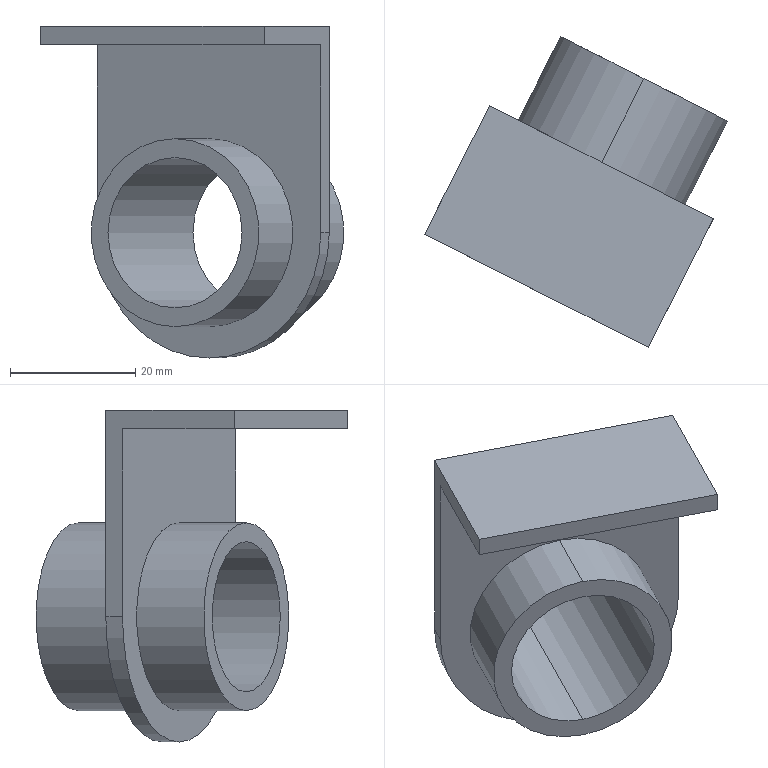Component | SolidWorks | ScribingMechanismAssembly-1_ScribingPlateFixedSleeve-1 | 1 solid | 17 faces | box 48.4 x 49.72 x 53 mm | volume 13758 mm3 | plane 9 | cylinder 8 | commonest cylinder face diameters 30 x4 24 x2 40 x2
STEP:
#1=COLOUR_RGB('',0.7922,0.8196,0.9333);
#2=FILL_AREA_STYLE_COLOUR('',#1);
#3=FILL_AREA_STYLE('',(#2));
#4=SURFACE_STYLE_FILL_AREA(#3);
#5=SURFACE_SIDE_STYLE('',(#4));
#6=SURFACE_STYLE_USAGE(.BOTH.,#5);
#7=PRESENTATION_STYLE_ASSIGNMENT((#6));
#8=CARTESIAN_POINT('',(-11.093,-16.169,37.952));
#9=VERTEX_POINT('',#8);
#10=CARTESIAN_POINT('',(-11.093,-16.169,36.771));
#11=VERTEX_POINT('',#10);
#12=CARTESIAN_POINT('',(-11.093,-16.169,37.361));
#13=DIRECTION('',(0.4521,0.892,0.));
#14=DIRECTION('',(-0.,-0.,1.));
#15=AXIS2_PLACEMENT_3D('',#12,#13,#14);
#16=CIRCLE('',#15,0.5906);
#17=EDGE_CURVE('',#9,#11,#16,.T.);
#18=ORIENTED_EDGE('',*,*,#17,.F.);
#19=CARTESIAN_POINT('',(-11.36,-16.696,37.952));
#20=VERTEX_POINT('',#19);
#21=CARTESIAN_POINT('',(-11.093,-16.169,37.952));
#22=DIRECTION('',(-0.4521,-0.892,-0.));
#23=VECTOR('',#22,39.37);
#24=LINE('',#21,#23);
#25=EDGE_CURVE('',#9,#20,#24,.T.);
#26=ORIENTED_EDGE('',*,*,#25,.T.);
#27=CARTESIAN_POINT('',(-11.36,-16.696,36.771));
#28=VERTEX_POINT('',#27);
#29=CARTESIAN_POINT('',(-11.36,-16.696,37.361));
#30=DIRECTION('',(-0.4521,-0.892,-0.));
#31=DIRECTION('',(0.892,-0.4521,-0.));
#32=AXIS2_PLACEMENT_3D('',#29,#30,#31);
#33=CIRCLE('',#32,0.5906);
#34=EDGE_CURVE('',#28,#20,#33,.T.);
#35=ORIENTED_EDGE('',*,*,#34,.F.);
#36=CARTESIAN_POINT('',(-11.093,-16.169,36.771));
#37=DIRECTION('',(-0.4521,-0.892,-0.));
#38=VECTOR('',#37,39.37);
#39=LINE('',#36,#38);
#40=EDGE_CURVE('',#11,#28,#39,.T.);
#41=ORIENTED_EDGE('',*,*,#40,.F.);
#42=EDGE_LOOP('',(#18,#26,#35,#41));
#43=FACE_OUTER_BOUND('',#42,.T.);
#44=CARTESIAN_POINT('',(-11.093,-16.169,37.361));
#45=DIRECTION('',(-0.4521,-0.892,-0.));
#46=DIRECTION('',(0.,0.,-1.));
#47=AXIS2_PLACEMENT_3D('',#44,#45,#46);
#48=CYLINDRICAL_SURFACE('',#47,0.5906);
#49=ADVANCED_FACE('',(#43),#48,.T.);
#50=CARTESIAN_POINT('',(-11.627,-17.223,36.889));
#51=VERTEX_POINT('',#50);
#52=CARTESIAN_POINT('',(-11.627,-17.223,37.834));
#53=VERTEX_POINT('',#52);
#54=CARTESIAN_POINT('',(-11.627,-17.223,37.361));
#55=DIRECTION('',(0.4521,0.892,0.));
#56=DIRECTION('',(-0.,-0.,1.));
#57=AXIS2_PLACEMENT_3D('',#54,#55,#56);
#58=CIRCLE('',#57,0.4724);
#59=EDGE_CURVE('',#51,#53,#58,.T.);
#60=ORIENTED_EDGE('',*,*,#59,.F.);
#61=CARTESIAN_POINT('',(-11.093,-16.169,36.889));
#62=VERTEX_POINT('',#61);
#63=CARTESIAN_POINT('',(-11.538,-17.047,36.889));
#64=DIRECTION('',(0.4521,0.892,0.));
#65=VECTOR('',#64,39.37);
#66=LINE('',#63,#65);
#67=EDGE_CURVE('',#51,#62,#66,.T.);
#68=ORIENTED_EDGE('',*,*,#67,.T.);
#69=CARTESIAN_POINT('',(-11.093,-16.169,37.834));
#70=VERTEX_POINT('',#69);
#71=CARTESIAN_POINT('',(-11.093,-16.169,37.361));
#72=DIRECTION('',(0.4521,0.892,0.));
#73=DIRECTION('',(-0.,-0.,1.));
#74=AXIS2_PLACEMENT_3D('',#71,#72,#73);
#75=CIRCLE('',#74,0.4724);
#76=EDGE_CURVE('',#62,#70,#75,.T.);
#77=ORIENTED_EDGE('',*,*,#76,.T.);
#78=CARTESIAN_POINT('',(-11.538,-17.047,37.834));
#79=DIRECTION('',(0.4521,0.892,0.));
#80=VECTOR('',#79,39.37);
#81=LINE('',#78,#80);
#82=EDGE_CURVE('',#53,#70,#81,.T.);
#83=ORIENTED_EDGE('',*,*,#82,.F.);
#84=EDGE_LOOP('',(#60,#68,#77,#83));
#85=FACE_OUTER_BOUND('',#84,.T.);
#86=CARTESIAN_POINT('',(-11.538,-17.047,37.361));
#87=DIRECTION('',(0.4521,0.892,0.));
#88=DIRECTION('',(-0.,-0.,1.));
#89=AXIS2_PLACEMENT_3D('',#86,#87,#88);
#90=CYLINDRICAL_SURFACE('',#89,0.4724);
#91=ADVANCED_FACE('',(#85),#90,.F.);
#92=CARTESIAN_POINT('',(-11.413,-16.801,36.771));
#93=VERTEX_POINT('',#92);
#94=CARTESIAN_POINT('',(-11.413,-16.801,37.952));
#95=VERTEX_POINT('',#94);
#96=CARTESIAN_POINT('',(-11.413,-16.801,37.361));
#97=DIRECTION('',(-0.4521,-0.892,-0.));
#98=DIRECTION('',(0.892,-0.4521,-0.));
#99=AXIS2_PLACEMENT_3D('',#96,#97,#98);
#100=CIRCLE('',#99,0.5906);
#101=EDGE_CURVE('',#93,#95,#100,.T.);
#102=ORIENTED_EDGE('',*,*,#101,.T.);
#103=CARTESIAN_POINT('',(-11.627,-17.223,37.952));
#104=VERTEX_POINT('',#103);
#105=CARTESIAN_POINT('',(-11.093,-16.169,37.952));
#106=DIRECTION('',(-0.4521,-0.892,-0.));
#107=VECTOR('',#106,39.37);
#108=LINE('',#105,#107);
#109=EDGE_CURVE('',#95,#104,#108,.T.);
#110=ORIENTED_EDGE('',*,*,#109,.T.);
#111=CARTESIAN_POINT('',(-11.627,-17.223,36.771));
#112=VERTEX_POINT('',#111);
#113=CARTESIAN_POINT('',(-11.627,-17.223,37.361));
#114=DIRECTION('',(0.4521,0.892,0.));
#115=DIRECTION('',(-0.,-0.,1.));
#116=AXIS2_PLACEMENT_3D('',#113,#114,#115);
#117=CIRCLE('',#116,0.5906);
#118=EDGE_CURVE('',#104,#112,#117,.T.);
#119=ORIENTED_EDGE('',*,*,#118,.T.);
#120=CARTESIAN_POINT('',(-11.093,-16.169,36.771));
#121=DIRECTION('',(-0.4521,-0.892,-0.));
#122=VECTOR('',#121,39.37);
#123=LINE('',#120,#122);
#124=EDGE_CURVE('',#93,#112,#123,.T.);
#125=ORIENTED_EDGE('',*,*,#124,.F.);
#126=EDGE_LOOP('',(#102,#110,#119,#125));
#127=FACE_OUTER_BOUND('',#126,.T.);
#128=CARTESIAN_POINT('',(-11.093,-16.169,37.361));
#129=DIRECTION('',(-0.4521,-0.892,-0.));
#130=DIRECTION('',(0.,0.,-1.));
#131=AXIS2_PLACEMENT_3D('',#128,#129,#130);
#132=CYLINDRICAL_SURFACE('',#131,0.5906);
#133=ADVANCED_FACE('',(#127),#132,.T.);
#134=CARTESIAN_POINT('',(-10.657,-17.052,37.361));
#135=VERTEX_POINT('',#134);
#136=CARTESIAN_POINT('',(-11.36,-16.696,36.574));
#137=VERTEX_POINT('',#136);
#138=CARTESIAN_POINT('',(-11.36,-16.696,37.361));
#139=DIRECTION('',(0.4521,0.892,0.));
#140=DIRECTION('',(0.892,-0.4521,-0.));
#141=AXIS2_PLACEMENT_3D('',#138,#139,#140);
#142=CIRCLE('',#141,0.7874);
#143=EDGE_CURVE('',#135,#137,#142,.T.);
#144=ORIENTED_EDGE('',*,*,#143,.T.);
#145=CARTESIAN_POINT('',(-12.062,-16.34,37.361));
#146=VERTEX_POINT('',#145);
#147=CARTESIAN_POINT('',(-11.36,-16.696,37.361));
#148=DIRECTION('',(0.4521,0.892,0.));
#149=DIRECTION('',(0.892,-0.4521,-0.));
#150=AXIS2_PLACEMENT_3D('',#147,#148,#149);
#151=CIRCLE('',#150,0.7874);
#152=EDGE_CURVE('',#137,#146,#151,.T.);
#153=ORIENTED_EDGE('',*,*,#152,.T.);
#154=CARTESIAN_POINT('',(-12.062,-16.34,38.66));
#155=VERTEX_POINT('',#154);
#156=CARTESIAN_POINT('',(-12.062,-16.34,38.542));
#157=DIRECTION('',(0.,0.,-1.));
#158=VECTOR('',#157,39.37);
#159=LINE('',#156,#158);
#160=EDGE_CURVE('',#155,#146,#159,.T.);
#161=ORIENTED_EDGE('',*,*,#160,.F.);
#162=CARTESIAN_POINT('',(-10.657,-17.052,38.66));
#163=VERTEX_POINT('',#162);
#164=CARTESIAN_POINT('',(-10.657,-17.052,38.66));
#165=DIRECTION('',(-0.892,0.4521,0.));
#166=VECTOR('',#165,39.37);
#167=LINE('',#164,#166);
#168=EDGE_CURVE('',#163,#155,#167,.T.);
#169=ORIENTED_EDGE('',*,*,#168,.F.);
#170=CARTESIAN_POINT('',(-10.657,-17.052,38.148));
#171=DIRECTION('',(0.,0.,-1.));
#172=VECTOR('',#171,39.37);
#173=LINE('',#170,#172);
#174=EDGE_CURVE('',#163,#135,#173,.T.);
#175=ORIENTED_EDGE('',*,*,#174,.T.);
#176=EDGE_LOOP('',(#144,#153,#161,#169,#175));
#177=FACE_OUTER_BOUND('',#176,.T.);
#178=ORIENTED_EDGE('',*,*,#34,.T.);
#179=CARTESIAN_POINT('',(-11.36,-16.696,37.361));
#180=DIRECTION('',(-0.4521,-0.892,-0.));
#181=DIRECTION('',(0.892,-0.4521,-0.));
#182=AXIS2_PLACEMENT_3D('',#179,#180,#181);
#183=CIRCLE('',#182,0.5906);
#184=EDGE_CURVE('',#20,#28,#183,.T.);
#185=ORIENTED_EDGE('',*,*,#184,.T.);
#186=EDGE_LOOP('',(#178,#185));
#187=FACE_BOUND('',#186,.T.);
#188=CARTESIAN_POINT('',(-10.657,-17.052,38.542));
#189=DIRECTION('',(0.4521,0.892,0.));
#190=DIRECTION('',(0.892,-0.4521,-0.));
#191=AXIS2_PLACEMENT_3D('',#188,#189,#190);
#192=PLANE('',#191);
#193=ADVANCED_FACE('',(#177,#187),#192,.T.);
#194=CARTESIAN_POINT('',(-12.115,-16.445,38.542));
#195=VERTEX_POINT('',#194);
#196=CARTESIAN_POINT('',(-12.115,-16.445,37.361));
#197=VERTEX_POINT('',#196);
#198=CARTESIAN_POINT('',(-12.115,-16.445,38.542));
#199=DIRECTION('',(0.,0.,-1.));
#200=VECTOR('',#199,39.37);
#201=LINE('',#198,#200);
#202=EDGE_CURVE('',#195,#197,#201,.T.);
#203=ORIENTED_EDGE('',*,*,#202,.T.);
#204=CARTESIAN_POINT('',(-11.413,-16.801,36.574));
#205=VERTEX_POINT('',#204);
#206=CARTESIAN_POINT('',(-11.413,-16.801,37.361));
#207=DIRECTION('',(-0.4521,-0.892,-0.));
#208=DIRECTION('',(0.892,-0.4521,-0.));
#209=AXIS2_PLACEMENT_3D('',#206,#207,#208);
#210=CIRCLE('',#209,0.7874);
#211=EDGE_CURVE('',#197,#205,#210,.T.);
#212=ORIENTED_EDGE('',*,*,#211,.T.);
#213=CARTESIAN_POINT('',(-10.711,-17.157,37.361));
#214=VERTEX_POINT('',#213);
#215=CARTESIAN_POINT('',(-11.413,-16.801,37.361));
#216=DIRECTION('',(-0.4521,-0.892,-0.));
#217=DIRECTION('',(0.892,-0.4521,-0.));
#218=AXIS2_PLACEMENT_3D('',#215,#216,#217);
#219=CIRCLE('',#218,0.7874);
#220=EDGE_CURVE('',#205,#214,#219,.T.);
#221=ORIENTED_EDGE('',*,*,#220,.T.);
#222=CARTESIAN_POINT('',(-10.711,-17.157,38.542));
#223=VERTEX_POINT('',#222);
#224=CARTESIAN_POINT('',(-10.711,-17.157,38.148));
#225=DIRECTION('',(0.,0.,-1.));
#226=VECTOR('',#225,39.37);
#227=LINE('',#224,#226);
#228=EDGE_CURVE('',#223,#214,#227,.T.);
#229=ORIENTED_EDGE('',*,*,#228,.F.);
#230=CARTESIAN_POINT('',(-10.711,-17.157,38.542));
#231=DIRECTION('',(-0.892,0.4521,0.));
#232=VECTOR('',#231,39.37);
#233=LINE('',#230,#232);
#234=EDGE_CURVE('',#223,#195,#233,.T.);
#235=ORIENTED_EDGE('',*,*,#234,.T.);
#236=EDGE_LOOP('',(#203,#212,#221,#229,#235));
#237=FACE_OUTER_BOUND('',#236,.T.);
#238=ORIENTED_EDGE('',*,*,#101,.F.);
#239=CARTESIAN_POINT('',(-11.413,-16.801,37.361));
#240=DIRECTION('',(-0.4521,-0.892,-0.));
#241=DIRECTION('',(0.892,-0.4521,-0.));
#242=AXIS2_PLACEMENT_3D('',#239,#240,#241);
#243=CIRCLE('',#242,0.5906);
#244=EDGE_CURVE('',#95,#93,#243,.T.);
#245=ORIENTED_EDGE('',*,*,#244,.F.);
#246=EDGE_LOOP('',(#238,#245));
#247=FACE_BOUND('',#246,.T.);
#248=CARTESIAN_POINT('',(-10.711,-17.157,38.542));
#249=DIRECTION('',(0.4521,0.892,0.));
#250=DIRECTION('',(0.892,-0.4521,-0.));
#251=AXIS2_PLACEMENT_3D('',#248,#249,#250);
#252=PLANE('',#251);
#253=ADVANCED_FACE('',(#237,#247),#252,.F.);
#254=CARTESIAN_POINT('',(-12.471,-17.148,38.66));
#255=VERTEX_POINT('',#254);
#256=CARTESIAN_POINT('',(-12.471,-17.148,38.66));
#257=DIRECTION('',(0.4521,0.892,0.));
#258=VECTOR('',#257,39.37);
#259=LINE('',#256,#258);
#260=EDGE_CURVE('',#255,#155,#259,.T.);
#261=ORIENTED_EDGE('',*,*,#260,.F.);
#262=CARTESIAN_POINT('',(-11.067,-17.86,38.66));
#263=VERTEX_POINT('',#262);
#264=CARTESIAN_POINT('',(-11.067,-17.86,38.66));
#265=DIRECTION('',(-0.892,0.4521,0.));
#266=VECTOR('',#265,39.37);
#267=LINE('',#264,#266);
#268=EDGE_CURVE('',#263,#255,#267,.T.);
#269=ORIENTED_EDGE('',*,*,#268,.F.);
#270=CARTESIAN_POINT('',(-11.067,-17.86,38.66));
#271=DIRECTION('',(0.4521,0.892,0.));
#272=VECTOR('',#271,39.37);
#273=LINE('',#270,#272);
#274=EDGE_CURVE('',#263,#163,#273,.T.);
#275=ORIENTED_EDGE('',*,*,#274,.T.);
#276=ORIENTED_EDGE('',*,*,#168,.T.);
#277=EDGE_LOOP('',(#261,#269,#275,#276));
#278=FACE_OUTER_BOUND('',#277,.T.);
#279=CARTESIAN_POINT('',(-11.067,-17.86,38.66));
#280=DIRECTION('',(-0.,-0.,1.));
#281=DIRECTION('',(0.892,-0.4521,-0.));
#282=AXIS2_PLACEMENT_3D('',#279,#280,#281);
#283=PLANE('',#282);
#284=ADVANCED_FACE('',(#278),#283,.T.);
#285=CARTESIAN_POINT('',(-12.471,-17.148,38.542));
#286=VERTEX_POINT('',#285);
#287=CARTESIAN_POINT('',(-12.471,-17.148,38.542));
#288=DIRECTION('',(-0.,-0.,1.));
#289=VECTOR('',#288,39.37);
#290=LINE('',#287,#289);
#291=EDGE_CURVE('',#286,#255,#290,.T.);
#292=ORIENTED_EDGE('',*,*,#291,.F.);
#293=CARTESIAN_POINT('',(-11.067,-17.86,38.542));
#294=VERTEX_POINT('',#293);
#295=CARTESIAN_POINT('',(-11.067,-17.86,38.542));
#296=DIRECTION('',(-0.892,0.4521,0.));
#297=VECTOR('',#296,39.37);
#298=LINE('',#295,#297);
#299=EDGE_CURVE('',#294,#286,#298,.T.);
#300=ORIENTED_EDGE('',*,*,#299,.F.);
#301=CARTESIAN_POINT('',(-11.067,-17.86,38.542));
#302=DIRECTION('',(-0.,-0.,1.));
#303=VECTOR('',#302,39.37);
#304=LINE('',#301,#303);
#305=EDGE_CURVE('',#294,#263,#304,.T.);
#306=ORIENTED_EDGE('',*,*,#305,.T.);
#307=ORIENTED_EDGE('',*,*,#268,.T.);
#308=EDGE_LOOP('',(#292,#300,#306,#307));
#309=FACE_OUTER_BOUND('',#308,.T.);
#310=CARTESIAN_POINT('',(-11.067,-17.86,38.542));
#311=DIRECTION('',(-0.4521,-0.892,-0.));
#312=DIRECTION('',(-0.892,0.4521,0.));
#313=AXIS2_PLACEMENT_3D('',#310,#311,#312);
#314=PLANE('',#313);
#315=ADVANCED_FACE('',(#309),#314,.T.);
#316=CARTESIAN_POINT('',(-12.471,-17.148,38.542));
#317=DIRECTION('',(0.4521,0.892,0.));
#318=VECTOR('',#317,39.37);
#319=LINE('',#316,#318);
#320=EDGE_CURVE('',#286,#195,#319,.T.);
#321=ORIENTED_EDGE('',*,*,#320,.T.);
#322=ORIENTED_EDGE('',*,*,#234,.F.);
#323=CARTESIAN_POINT('',(-11.067,-17.86,38.542));
#324=DIRECTION('',(0.4521,0.892,0.));
#325=VECTOR('',#324,39.37);
#326=LINE('',#323,#325);
#327=EDGE_CURVE('',#294,#223,#326,.T.);
#328=ORIENTED_EDGE('',*,*,#327,.F.);
#329=ORIENTED_EDGE('',*,*,#299,.T.);
#330=EDGE_LOOP('',(#321,#322,#328,#329));
#331=FACE_OUTER_BOUND('',#330,.T.);
#332=CARTESIAN_POINT('',(-11.067,-17.86,38.542));
#333=DIRECTION('',(-0.,-0.,1.));
#334=DIRECTION('',(0.892,-0.4521,-0.));
#335=AXIS2_PLACEMENT_3D('',#332,#333,#334);
#336=PLANE('',#335);
#337=ADVANCED_FACE('',(#331),#336,.F.);
#338=ORIENTED_EDGE('',*,*,#228,.T.);
#339=CARTESIAN_POINT('',(-10.657,-17.052,37.361));
#340=DIRECTION('',(0.4521,0.892,0.));
#341=VECTOR('',#340,39.37);
#342=LINE('',#339,#341);
#343=EDGE_CURVE('',#214,#135,#342,.T.);
#344=ORIENTED_EDGE('',*,*,#343,.T.);
#345=ORIENTED_EDGE('',*,*,#174,.F.);
#346=ORIENTED_EDGE('',*,*,#274,.F.);
#347=ORIENTED_EDGE('',*,*,#305,.F.);
#348=ORIENTED_EDGE('',*,*,#327,.T.);
#349=EDGE_LOOP('',(#338,#344,#345,#346,#347,#348));
#350=FACE_OUTER_BOUND('',#349,.T.);
#351=CARTESIAN_POINT('',(-11.067,-17.86,38.542));
#352=DIRECTION('',(-0.892,0.4521,0.));
#353=DIRECTION('',(-0.,-0.,1.));
#354=AXIS2_PLACEMENT_3D('',#351,#352,#353);
#355=PLANE('',#354);
#356=ADVANCED_FACE('',(#350),#355,.F.);
#357=ORIENTED_EDGE('',*,*,#160,.T.);
#358=CARTESIAN_POINT('',(-12.471,-17.148,37.361));
#359=DIRECTION('',(-0.4521,-0.892,-0.));
#360=VECTOR('',#359,39.37);
#361=LINE('',#358,#360);
#362=EDGE_CURVE('',#146,#197,#361,.T.);
#363=ORIENTED_EDGE('',*,*,#362,.T.);
#364=ORIENTED_EDGE('',*,*,#202,.F.);
#365=ORIENTED_EDGE('',*,*,#320,.F.);
#366=ORIENTED_EDGE('',*,*,#291,.T.);
#367=ORIENTED_EDGE('',*,*,#260,.T.);
#368=EDGE_LOOP('',(#357,#363,#364,#365,#366,#367));
#369=FACE_OUTER_BOUND('',#368,.T.);
#370=CARTESIAN_POINT('',(-12.471,-17.148,38.542));
#371=DIRECTION('',(-0.892,0.4521,0.));
#372=DIRECTION('',(-0.,-0.,1.));
#373=AXIS2_PLACEMENT_3D('',#370,#371,#372);
#374=PLANE('',#373);
#375=ADVANCED_FACE('',(#369),#374,.T.);
#376=CARTESIAN_POINT('',(-11.413,-16.801,36.574));
#377=DIRECTION('',(-0.4521,-0.892,-0.));
#378=VECTOR('',#377,39.37);
#379=LINE('',#376,#378);
#380=EDGE_CURVE('',#137,#205,#379,.T.);
#381=ORIENTED_EDGE('',*,*,#380,.F.);
#382=ORIENTED_EDGE('',*,*,#143,.F.);
#383=ORIENTED_EDGE('',*,*,#343,.F.);
#384=ORIENTED_EDGE('',*,*,#220,.F.);
#385=EDGE_LOOP('',(#381,#382,#383,#384));
#386=FACE_OUTER_BOUND('',#385,.T.);
#387=CARTESIAN_POINT('',(-11.36,-16.696,37.361));
#388=DIRECTION('',(0.4521,0.892,0.));
#389=DIRECTION('',(0.892,-0.4521,-0.));
#390=AXIS2_PLACEMENT_3D('',#387,#388,#389);
#391=CYLINDRICAL_SURFACE('',#390,0.7874);
#392=ADVANCED_FACE('',(#386),#391,.T.);
#393=ORIENTED_EDGE('',*,*,#152,.F.);
#394=ORIENTED_EDGE('',*,*,#380,.T.);
#395=ORIENTED_EDGE('',*,*,#211,.F.);
#396=ORIENTED_EDGE('',*,*,#362,.F.);
#397=EDGE_LOOP('',(#393,#394,#395,#396));
#398=FACE_OUTER_BOUND('',#397,.T.);
#399=CARTESIAN_POINT('',(-11.769,-17.504,37.361));
#400=DIRECTION('',(-0.4521,-0.892,-0.));
#401=DIRECTION('',(-0.892,0.4521,0.));
#402=AXIS2_PLACEMENT_3D('',#399,#400,#401);
#403=CYLINDRICAL_SURFACE('',#402,0.7874);
#404=ADVANCED_FACE('',(#398),#403,.T.);
#405=ORIENTED_EDGE('',*,*,#109,.F.);
#406=ORIENTED_EDGE('',*,*,#244,.T.);
#407=ORIENTED_EDGE('',*,*,#124,.T.);
#408=CARTESIAN_POINT('',(-11.627,-17.223,37.361));
#409=DIRECTION('',(0.4521,0.892,0.));
#410=DIRECTION('',(-0.,-0.,1.));
#411=AXIS2_PLACEMENT_3D('',#408,#409,#410);
#412=CIRCLE('',#411,0.5906);
#413=EDGE_CURVE('',#112,#104,#412,.T.);
#414=ORIENTED_EDGE('',*,*,#413,.T.);
#415=EDGE_LOOP('',(#405,#406,#407,#414));
#416=FACE_OUTER_BOUND('',#415,.T.);
#417=CARTESIAN_POINT('',(-11.093,-16.169,37.361));
#418=DIRECTION('',(-0.4521,-0.892,-0.));
#419=DIRECTION('',(0.,0.,-1.));
#420=AXIS2_PLACEMENT_3D('',#417,#418,#419);
#421=CYLINDRICAL_SURFACE('',#420,0.5906);
#422=ADVANCED_FACE('',(#416),#421,.T.);
#423=ORIENTED_EDGE('',*,*,#413,.F.);
#424=ORIENTED_EDGE('',*,*,#118,.F.);
#425=EDGE_LOOP('',(#423,#424));
#426=FACE_OUTER_BOUND('',#425,.T.);
#427=CARTESIAN_POINT('',(-11.627,-17.223,37.361));
#428=DIRECTION('',(0.4521,0.892,0.));
#429=DIRECTION('',(-0.,-0.,1.));
#430=AXIS2_PLACEMENT_3D('',#427,#428,#429);
#431=CIRCLE('',#430,0.4724);
#432=EDGE_CURVE('',#53,#51,#431,.T.);
#433=ORIENTED_EDGE('',*,*,#432,.T.);
#434=ORIENTED_EDGE('',*,*,#59,.T.);
#435=EDGE_LOOP('',(#433,#434));
#436=FACE_BOUND('',#435,.T.);
#437=CARTESIAN_POINT('',(-11.627,-17.223,37.361));
#438=DIRECTION('',(0.4521,0.892,0.));
#439=DIRECTION('',(-0.,-0.,1.));
#440=AXIS2_PLACEMENT_3D('',#437,#438,#439);
#441=PLANE('',#440);
#442=ADVANCED_FACE('',(#426,#436),#441,.F.);
#443=ORIENTED_EDGE('',*,*,#67,.F.);
#444=ORIENTED_EDGE('',*,*,#432,.F.);
#445=ORIENTED_EDGE('',*,*,#82,.T.);
#446=CARTESIAN_POINT('',(-11.093,-16.169,37.361));
#447=DIRECTION('',(0.4521,0.892,0.));
#448=DIRECTION('',(-0.,-0.,1.));
#449=AXIS2_PLACEMENT_3D('',#446,#447,#448);
#450=CIRCLE('',#449,0.4724);
#451=EDGE_CURVE('',#70,#62,#450,.T.);
#452=ORIENTED_EDGE('',*,*,#451,.T.);
#453=EDGE_LOOP('',(#443,#444,#445,#452));
#454=FACE_OUTER_BOUND('',#453,.T.);
#455=CARTESIAN_POINT('',(-11.538,-17.047,37.361));
#456=DIRECTION('',(0.4521,0.892,0.));
#457=DIRECTION('',(-0.,-0.,1.));
#458=AXIS2_PLACEMENT_3D('',#455,#456,#457);
#459=CYLINDRICAL_SURFACE('',#458,0.4724);
#460=ADVANCED_FACE('',(#454),#459,.F.);
#461=CARTESIAN_POINT('',(-11.093,-16.169,37.361));
#462=DIRECTION('',(0.4521,0.892,0.));
#463=DIRECTION('',(-0.,-0.,1.));
#464=AXIS2_PLACEMENT_3D('',#461,#462,#463);
#465=CIRCLE('',#464,0.5906);
#466=EDGE_CURVE('',#11,#9,#465,.T.);
#467=ORIENTED_EDGE('',*,*,#466,.T.);
#468=ORIENTED_EDGE('',*,*,#17,.T.);
#469=EDGE_LOOP('',(#467,#468));
#470=FACE_OUTER_BOUND('',#469,.T.);
#471=ORIENTED_EDGE('',*,*,#451,.F.);
#472=ORIENTED_EDGE('',*,*,#76,.F.);
#473=EDGE_LOOP('',(#471,#472));
#474=FACE_BOUND('',#473,.T.);
#475=CARTESIAN_POINT('',(-11.093,-16.169,37.361));
#476=DIRECTION('',(0.4521,0.892,0.));
#477=DIRECTION('',(-0.,-0.,1.));
#478=AXIS2_PLACEMENT_3D('',#475,#476,#477);
#479=PLANE('',#478);
#480=ADVANCED_FACE('',(#470,#474),#479,.T.);
#481=ORIENTED_EDGE('',*,*,#25,.F.);
#482=ORIENTED_EDGE('',*,*,#466,.F.);
#483=ORIENTED_EDGE('',*,*,#40,.T.);
#484=ORIENTED_EDGE('',*,*,#184,.F.);
#485=EDGE_LOOP('',(#481,#482,#483,#484));
#486=FACE_OUTER_BOUND('',#485,.T.);
#487=CARTESIAN_POINT('',(-11.093,-16.169,37.361));
#488=DIRECTION('',(-0.4521,-0.892,-0.));
#489=DIRECTION('',(0.,0.,-1.));
#490=AXIS2_PLACEMENT_3D('',#487,#488,#489);
#491=CYLINDRICAL_SURFACE('',#490,0.5906);
#492=ADVANCED_FACE('',(#486),#491,.T.);
#493=CLOSED_SHELL('',(#49,#91,#133,#193,#253,#284,#315,#337,#356,#375,#392,#404,#422,#442,#460,#480,#492));
#494=MANIFOLD_SOLID_BREP('',#493);
#495=STYLED_ITEM('',(#7),#494);
#496=(LENGTH_UNIT()NAMED_UNIT(*)SI_UNIT($,.METRE.));
#497=LENGTH_MEASURE_WITH_UNIT(LENGTH_MEASURE(0.0254),#496);
#498=DIMENSIONAL_EXPONENTS(1.,0.,0.,0.,0.,0.,0.);
#499=(CONVERSION_BASED_UNIT('',#497)LENGTH_UNIT()NAMED_UNIT(#498));
#500=UNCERTAINTY_MEASURE_WITH_UNIT(LENGTH_MEASURE(0.00001),#499,'','');
#501=(NAMED_UNIT(*)PLANE_ANGLE_UNIT()SI_UNIT($,.RADIAN.));
#502=(NAMED_UNIT(*)SI_UNIT($,.STERADIAN.)SOLID_ANGLE_UNIT());
#503=(GEOMETRIC_REPRESENTATION_CONTEXT(3)GLOBAL_UNCERTAINTY_ASSIGNED_CONTEXT((#500))GLOBAL_UNIT_ASSIGNED_CONTEXT((#499,#501,#502))REPRESENTATION_CONTEXT('',''));
#504=MECHANICAL_DESIGN_GEOMETRIC_PRESENTATION_REPRESENTATION('',(#495),#503);
#505=PRESENTATION_LAYER_ASSIGNMENT('','',(#495));
#506=CARTESIAN_POINT('',(0.,0.,0.));
#507=DIRECTION('',(0.,0.,1.));
#508=DIRECTION('',(1.,0.,0.));
#509=AXIS2_PLACEMENT_3D('',#506,#507,#508);
#510=(LENGTH_UNIT()NAMED_UNIT(*)SI_UNIT($,.METRE.));
#511=LENGTH_MEASURE_WITH_UNIT(LENGTH_MEASURE(0.0254),#510);
#512=DIMENSIONAL_EXPONENTS(1.,0.,0.,0.,0.,0.,0.);
#513=(CONVERSION_BASED_UNIT('',#511)LENGTH_UNIT()NAMED_UNIT(#512));
#514=UNCERTAINTY_MEASURE_WITH_UNIT(LENGTH_MEASURE(0.00001),#513,'','');
#515=(NAMED_UNIT(*)PLANE_ANGLE_UNIT()SI_UNIT($,.RADIAN.));
#516=(NAMED_UNIT(*)SI_UNIT($,.STERADIAN.)SOLID_ANGLE_UNIT());
#517=(GEOMETRIC_REPRESENTATION_CONTEXT(3)GLOBAL_UNCERTAINTY_ASSIGNED_CONTEXT((#514))GLOBAL_UNIT_ASSIGNED_CONTEXT((#513,#515,#516))REPRESENTATION_CONTEXT('',''));
#518=ADVANCED_BREP_SHAPE_REPRESENTATION('',(#494,#509),#517);